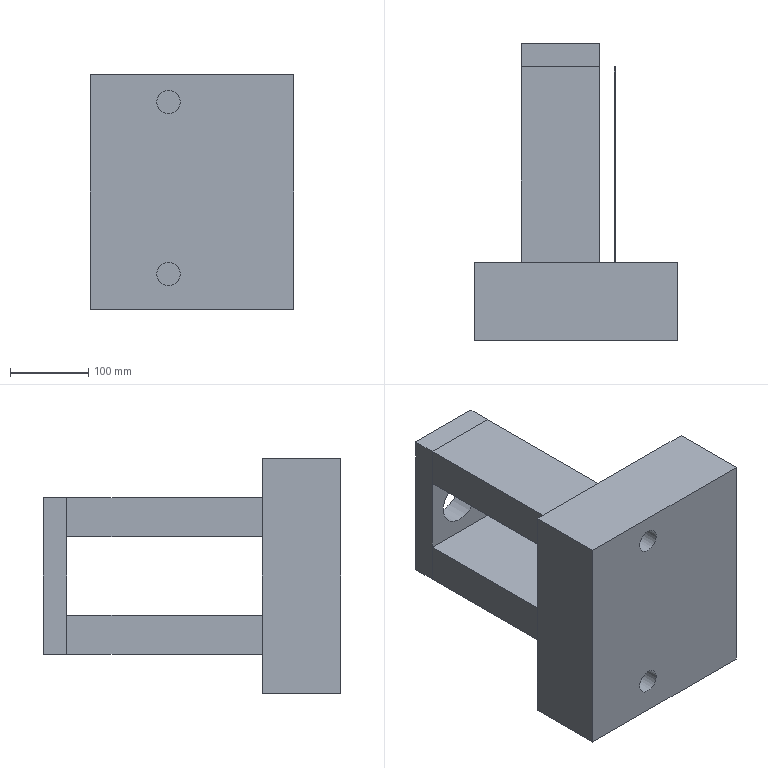Component | NX | LOWER_SUPPORT_SEAT | 2 solids | 31 faces | volume 10758658 mm3 | plane 28 | cylinder 3 | commonest cylinder face diameters 30 x2 60 x1